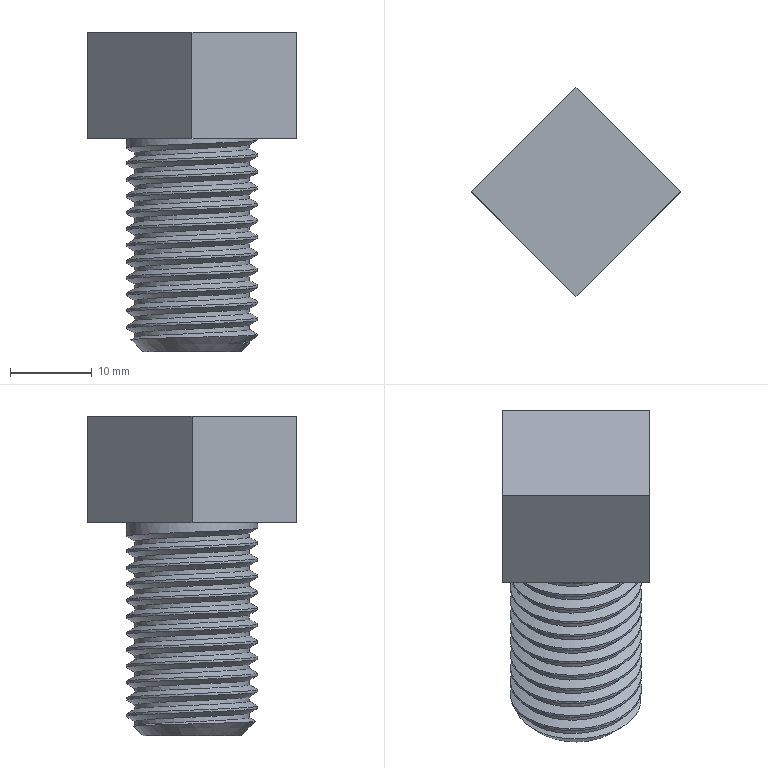Component | NX | SCREW | 1 solid | 15 faces | volume 9174 mm3 | plane 8 | spline 3 | cylinder 2 | cone 2 | commonest cylinder face diameters 16 x1 14 x1